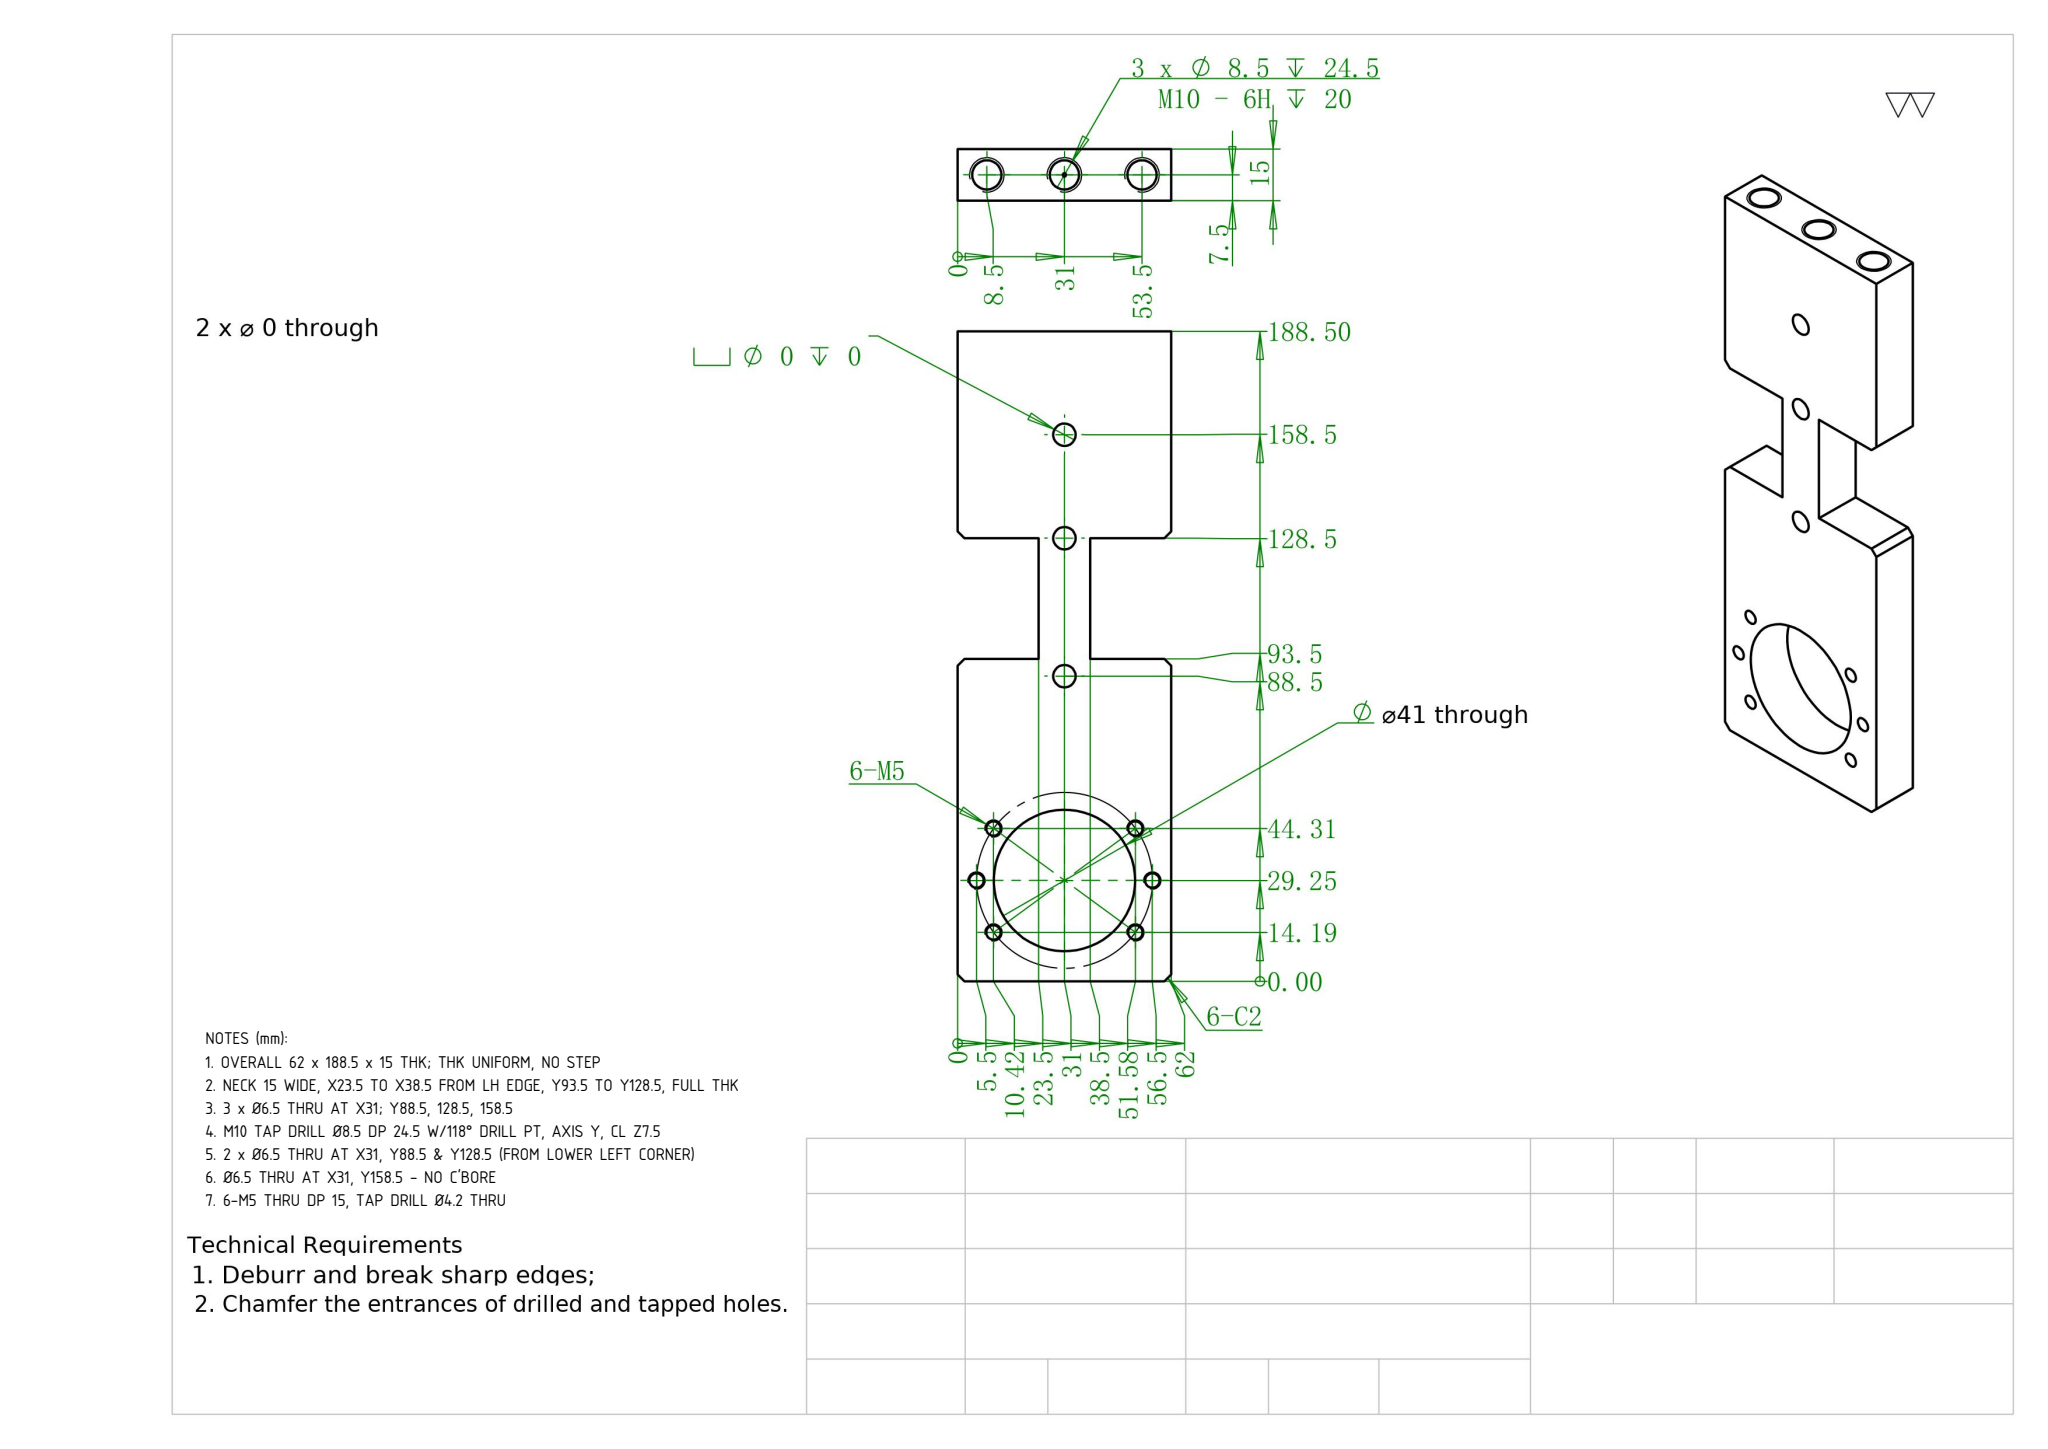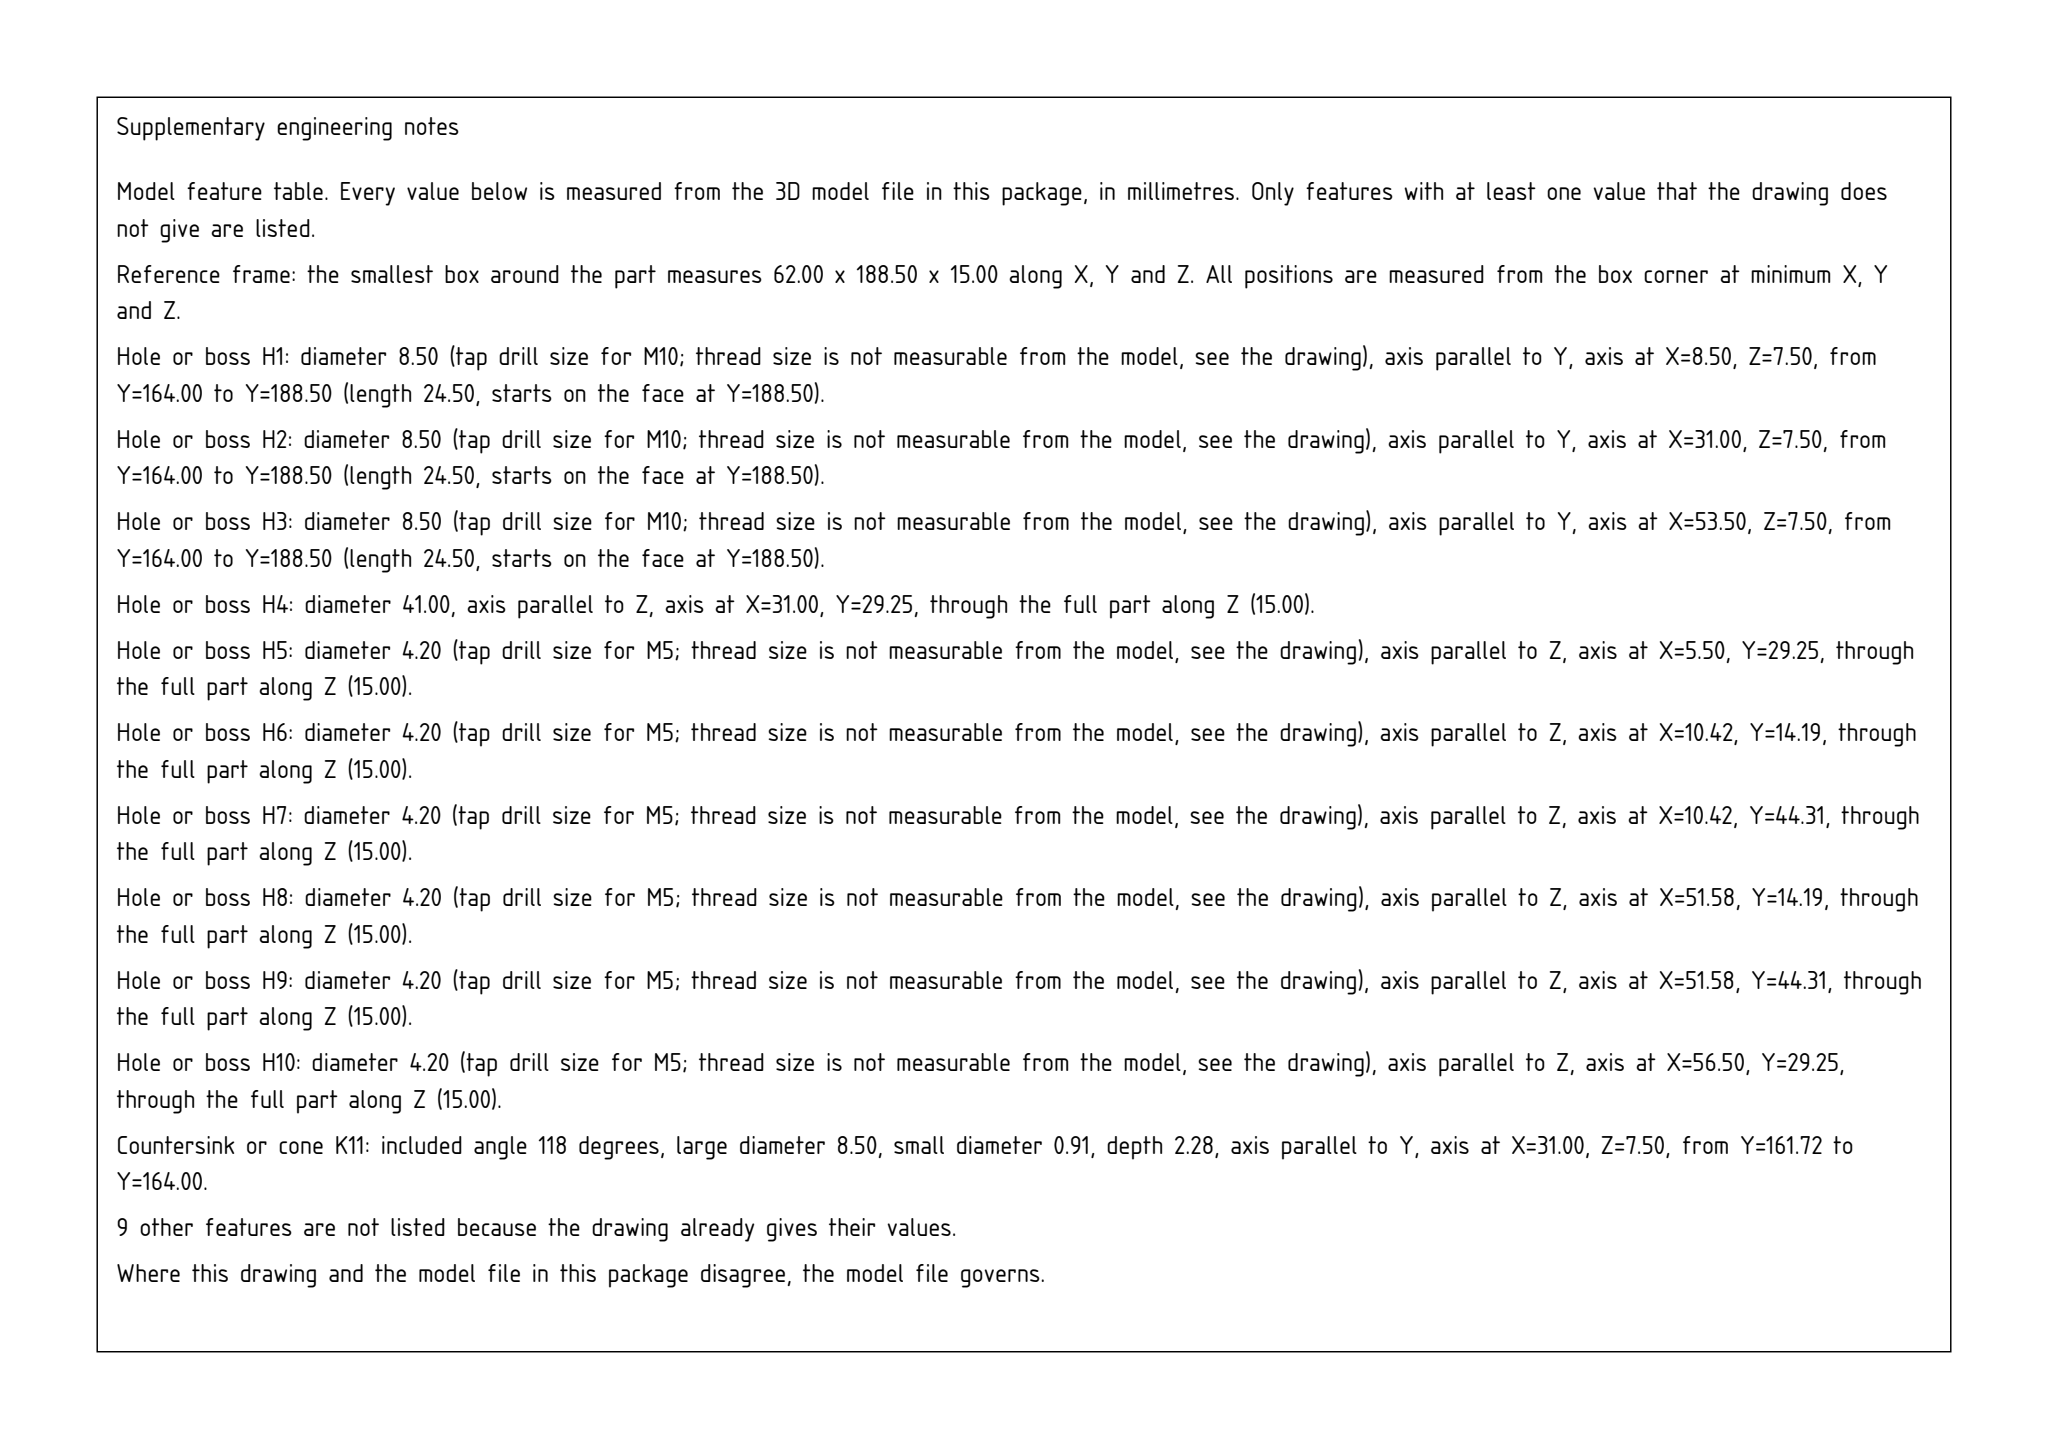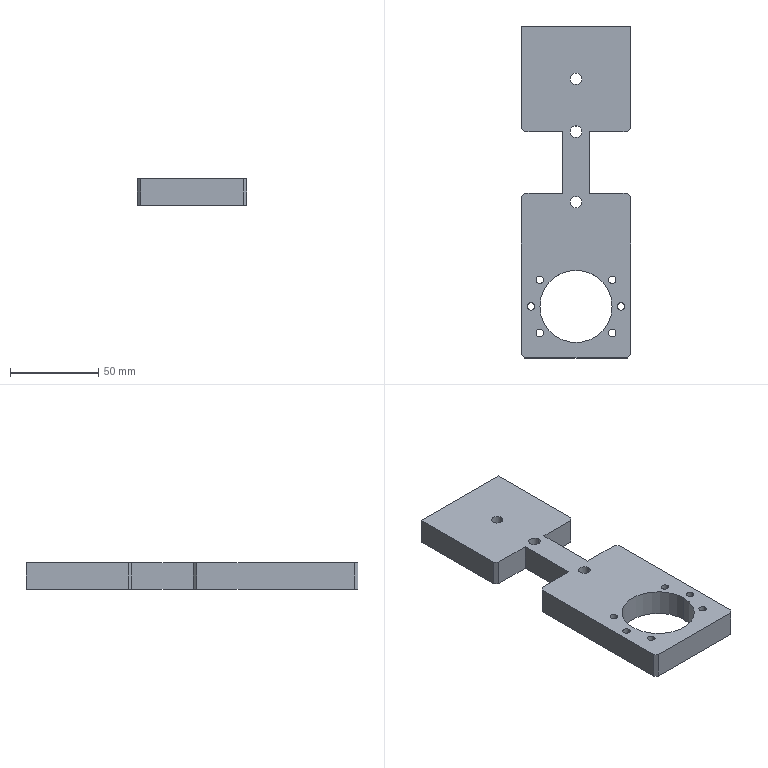Part | SolidWorks | mm | 1 solid | 52 faces | box 62 x 188.5 x 15 mm | volume 123590 mm3 | cylinder 26 | plane 20 | cone 6 | commonest cylinder face diameters 4.2 x12 6.5 x6 8.5 x6 41 x2
Drawing notes:
OVERALL 62 x 188.5 x 15 THK; THK UNIFORM, NO STEP | from the solid: bbox 62 x 188.5 x 15; only z planes 0.0 and 15.0; all z-cyl lengths 15.0
NECK 15 WIDE, X23.5 TO X38.5 FROM LH EDGE, Y93.5 TO Y128.5, FULL THK | from the solid: x planes 23.5 & 38.5; y planes 93.5 & 128.5; thk 15 thruout
3 x Ø6.5 THRU AT X31; Y88.5, 128.5, 158.5 | from the solid: cylinders dia 6.5 axis z at [31,88.5],[31,128.5],[31,158.5], length 15 = full thk
M10 TAP DRILL Ø8.5 DP 24.5 W/118° DRILL PT, AXIS Y, CL Z7.5 | from the solid: cylinders dia 8.5 axis y at z7.5, length 24.5; cones 118° ref dia 8.5
2 x Ø6.5 THRU AT X31, Y88.5 & Y128.5 (FROM LOWER LEFT CORNER) | from the solid: cylinders dia 6.5, axis z, pos [31,88.5] and [31,128.5], length 15 = full plate thk
Ø6.5 THRU AT X31, Y158.5 - NO C'BORE | from the solid: cylinder dia 6.5, axis z, pos [31,158.5], length 15 (thru); no counterbore feature in model
6-M5 THRU DP 15, TAP DRILL Ø4.2 THRU | from the solid: 6 x cylinders dia 4.2, axis z, length 15 = plate thk (z planes 0 and 15)
build123d program:
from build123d import *

# Parameters (mm, degrees)
SKETCH1_W                      = 62
SKETCH1_H                      = 188.5
SKETCH1_R                      = 20.5
BOSS_EXTRUDE1_DEPTH            = 15
M10_TAPPED_HOLE1_D             = 8.5
M10_TAPPED_HOLE1_DEPTH         = 24.5
M10_TAPPED_HOLE1_TIP           = 2.554
SKETCH5_W                      = 23.5
SKETCH5_H                      = 35
CUT_EXTRUDE1_DEPTH             = 101.345
CHAMFER1_SIZE                  = 2
CHAMFER2_SIZE                  = 2
M5_TAPPED_HOLE1_D              = 4.2
F_6_5_6_5_DIAMETER_HOLE1_D     = 6.5
F_6_5_6_5_DIAMETER_HOLE1_DEPTH = 15
F_6_5_6_5_DIAMETER_HOLE1_TIP   = 1.953
F_6_5_6_5_DIAMETER_HOLE2_D     = 6.5
F_6_5_6_5_DIAMETER_HOLE2_DEPTH = 15
F_6_5_6_5_DIAMETER_HOLE2_TIP   = 1.953


with BuildPart() as part:
    # Sketch1 → Boss-Extrude1 (new body)
    with BuildSketch(Plane.XY):
        Rectangle(SKETCH1_W, SKETCH1_H)
        with Locations((0, -65)):
            Circle(SKETCH1_R, mode=Mode.SUBTRACT)
    extrude(amount=BOSS_EXTRUDE1_DEPTH)

    # M10 Tapped Hole1
    with Locations(Plane(origin=(0, 94.25, 0), x_dir=(1, 0, 0), z_dir=(0, 1, 0))):
        with Locations((-22.5, -7.5), (0, -7.5), (22.5, -7.5)):
            Hole(M10_TAPPED_HOLE1_D / 2, depth=M10_TAPPED_HOLE1_DEPTH)
            with Locations((0, 0, -(M10_TAPPED_HOLE1_DEPTH + M10_TAPPED_HOLE1_TIP / 2))):  # 118° drill point
                Cone(0, M10_TAPPED_HOLE1_D / 2, M10_TAPPED_HOLE1_TIP, mode=Mode.SUBTRACT)

    # Sketch5 → Cut-Extrude1 (cut, through all)
    with BuildSketch(Plane.XY.offset(15)):
        with Locations((-19.25, 16.75)):
            Rectangle(SKETCH5_W, SKETCH5_H)
        with Locations((19.25, 16.75)):
            Rectangle(SKETCH5_W, SKETCH5_H)
    extrude(amount=-CUT_EXTRUDE1_DEPTH, mode=Mode.SUBTRACT)

    # Chamfer1
    chamfer1_edges = [part.edges().sort_by_distance(p)[0] for p in [
        (-31, -0.75, 7.5),
        (-31, 34.25, 7.5),
        (31, 34.25, 7.5),
        (31, -0.75, 7.5),
    ]]
    chamfer(chamfer1_edges, length=CHAMFER1_SIZE)

    # Chamfer2
    chamfer2_edges = [part.edges().sort_by_distance(p)[0] for p in [
        (31, -94.25, 7.5),
        (-31, -94.25, 7.5),
    ]]
    chamfer(chamfer2_edges, length=CHAMFER2_SIZE)

    # M5 Tapped Hole1 (through all)
    with Locations(Plane(origin=(0, 0, 0), x_dir=(-1, 0, 0), z_dir=(0, 0, -1))):
        with Locations((-25.5, -65), (-20.575, -80.063), (-20.575, -49.937), (20.575, -49.937), (20.575, -80.063), (25.5, -65)):
            Hole(M5_TAPPED_HOLE1_D / 2)

    # 6.5 _6.5_ Diameter Hole1
    with Locations(Plane.XY.offset(15)):
        with Locations((0, 64.25), (0, -5.75)):
            Hole(F_6_5_6_5_DIAMETER_HOLE1_D / 2, depth=F_6_5_6_5_DIAMETER_HOLE1_DEPTH)
            with Locations((0, 0, -(F_6_5_6_5_DIAMETER_HOLE1_DEPTH + F_6_5_6_5_DIAMETER_HOLE1_TIP / 2))):  # 118° drill point
                Cone(0, F_6_5_6_5_DIAMETER_HOLE1_D / 2, F_6_5_6_5_DIAMETER_HOLE1_TIP, mode=Mode.SUBTRACT)

    # 6.5 _6.5_ Diameter Hole2
    with Locations(Plane.XY.offset(15)):
        with Locations((0, 34.25)):
            Hole(F_6_5_6_5_DIAMETER_HOLE2_D / 2, depth=F_6_5_6_5_DIAMETER_HOLE2_DEPTH)
            with Locations((0, 0, -(F_6_5_6_5_DIAMETER_HOLE2_DEPTH + F_6_5_6_5_DIAMETER_HOLE2_TIP / 2))):  # 118° drill point
                Cone(0, F_6_5_6_5_DIAMETER_HOLE2_D / 2, F_6_5_6_5_DIAMETER_HOLE2_TIP, mode=Mode.SUBTRACT)


solid = part.part